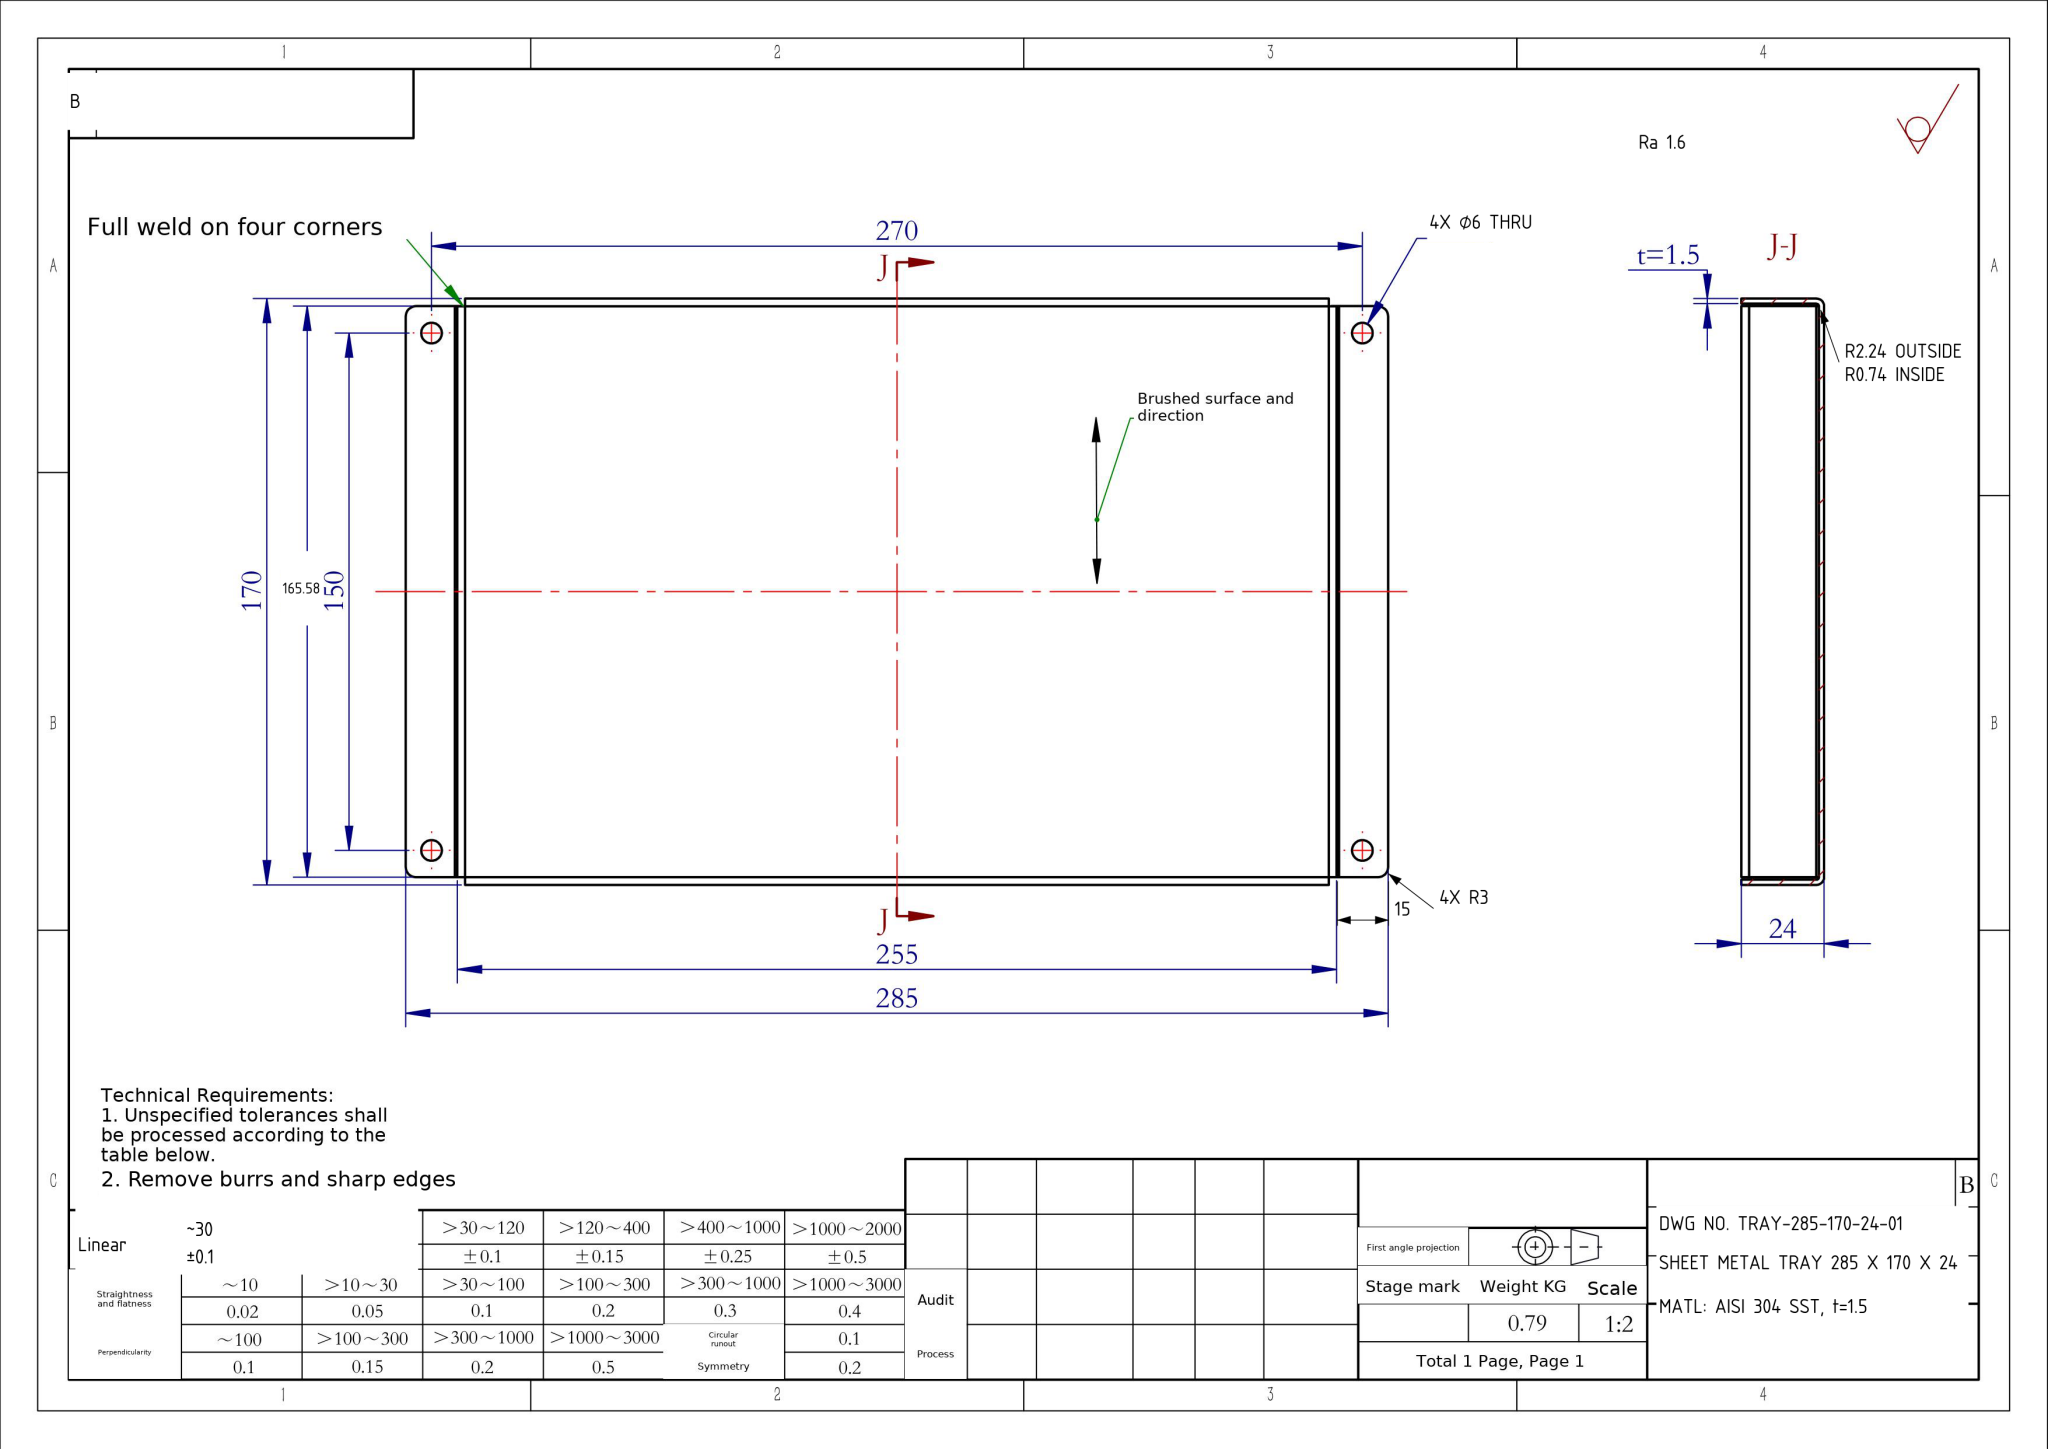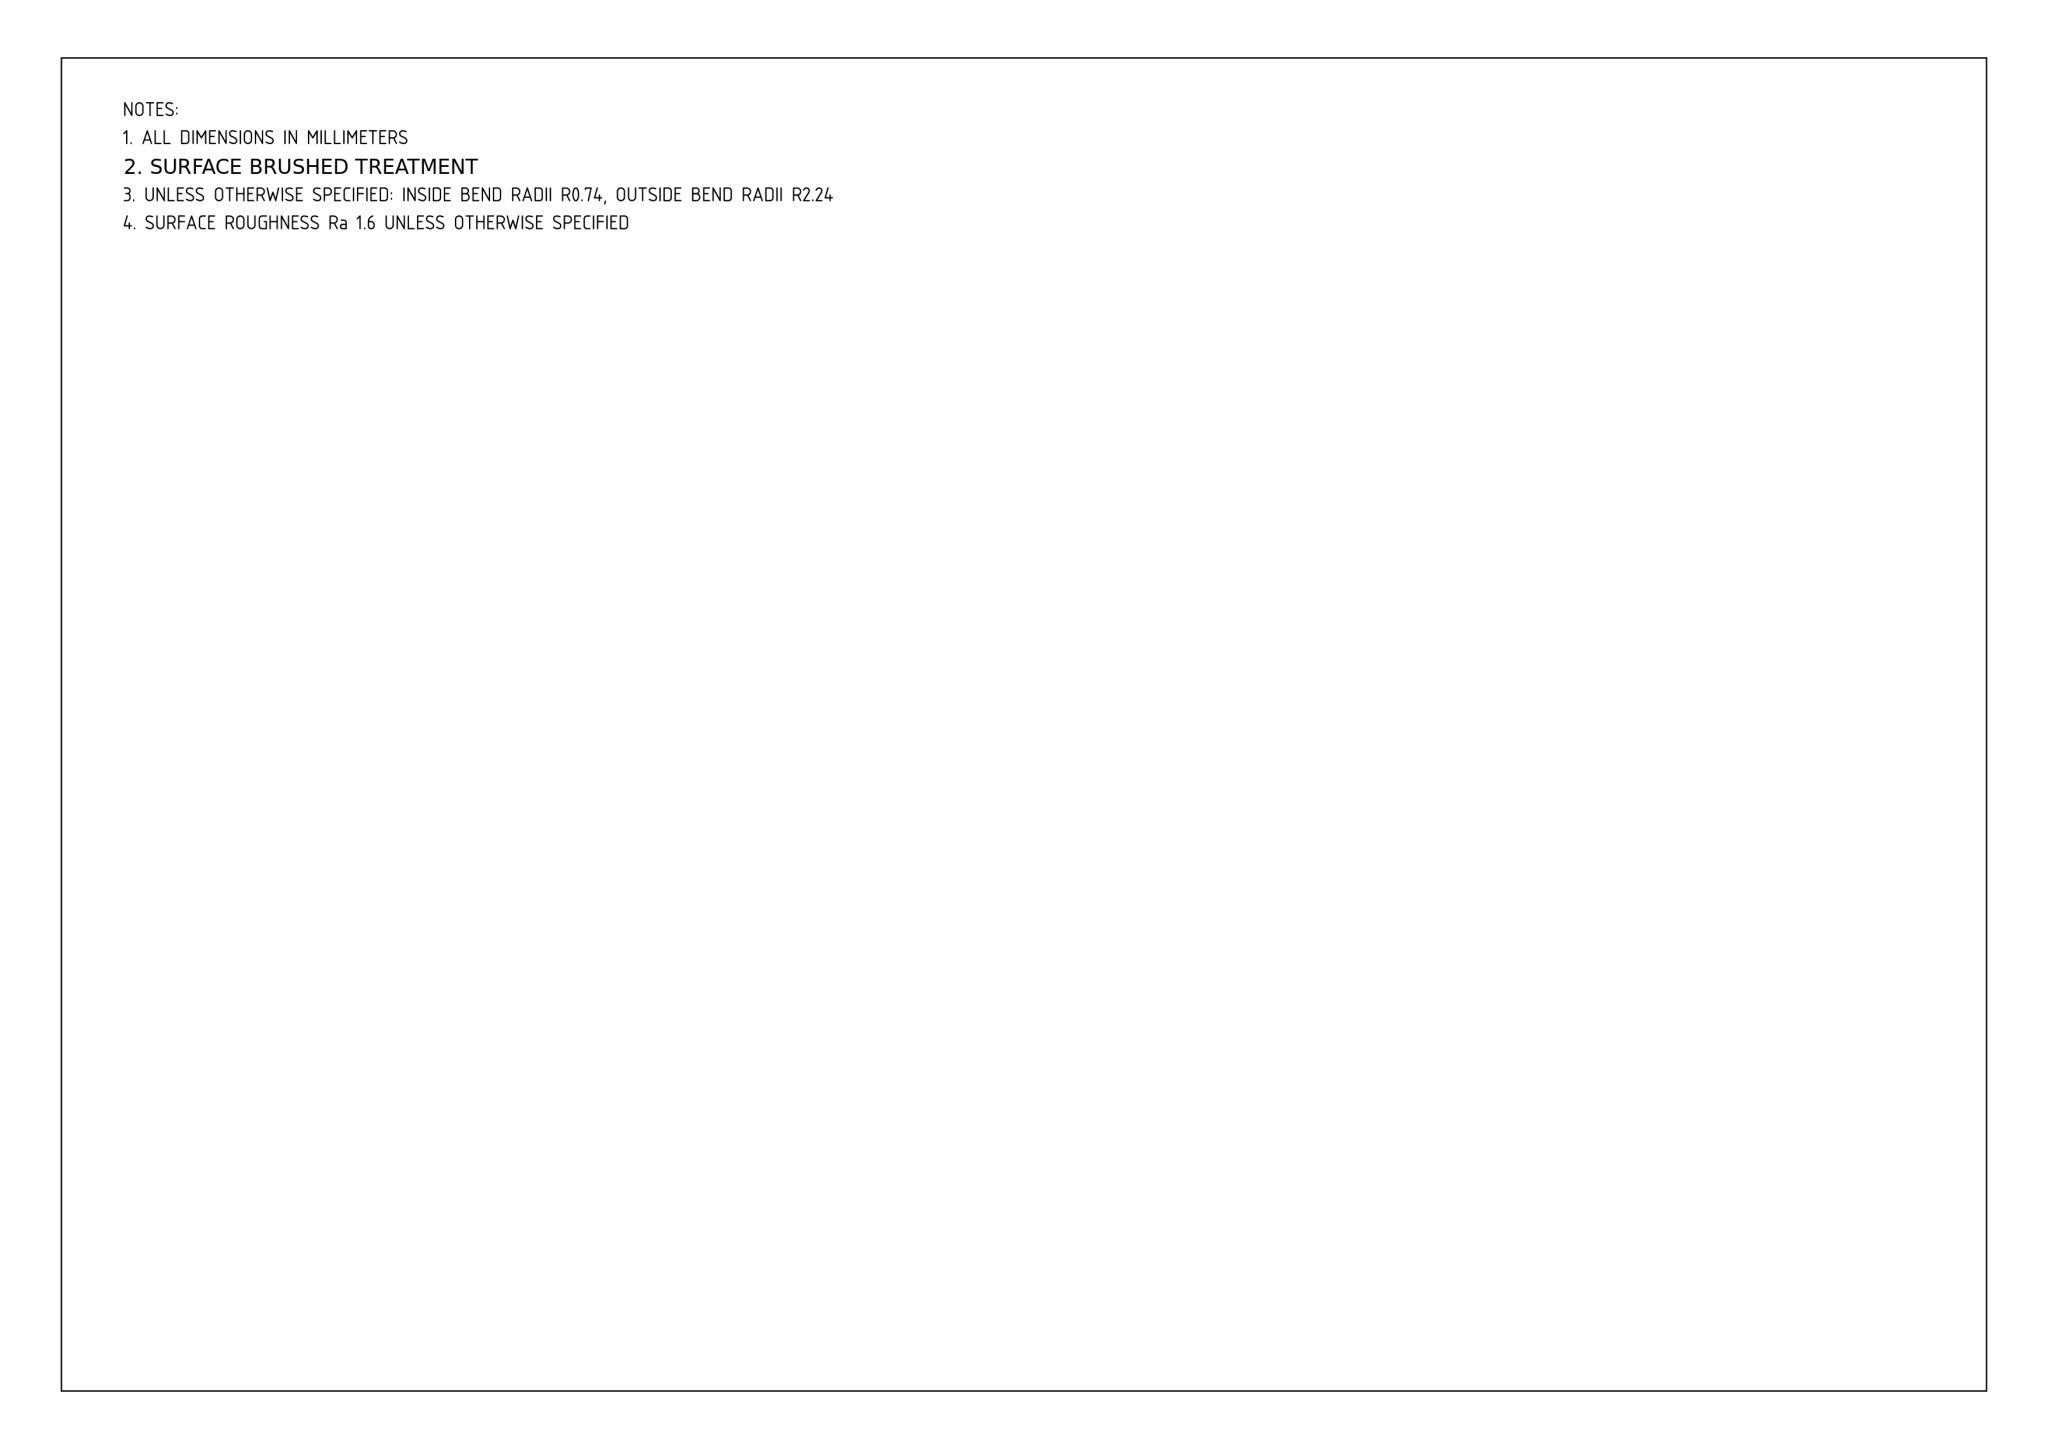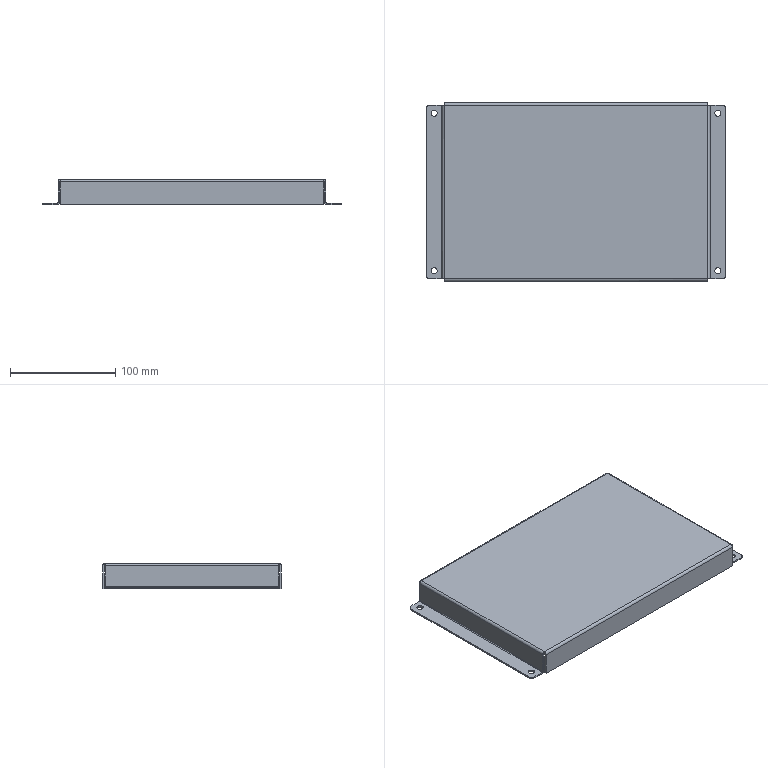Part | NX | mm | 1 solid | 66 faces | box 285 x 170 x 24 mm | volume 99244 mm3 | plane 34 | cylinder 24 | spline 8 | commonest cylinder face diameters 6 x12 4.473 x6 1.473 x6